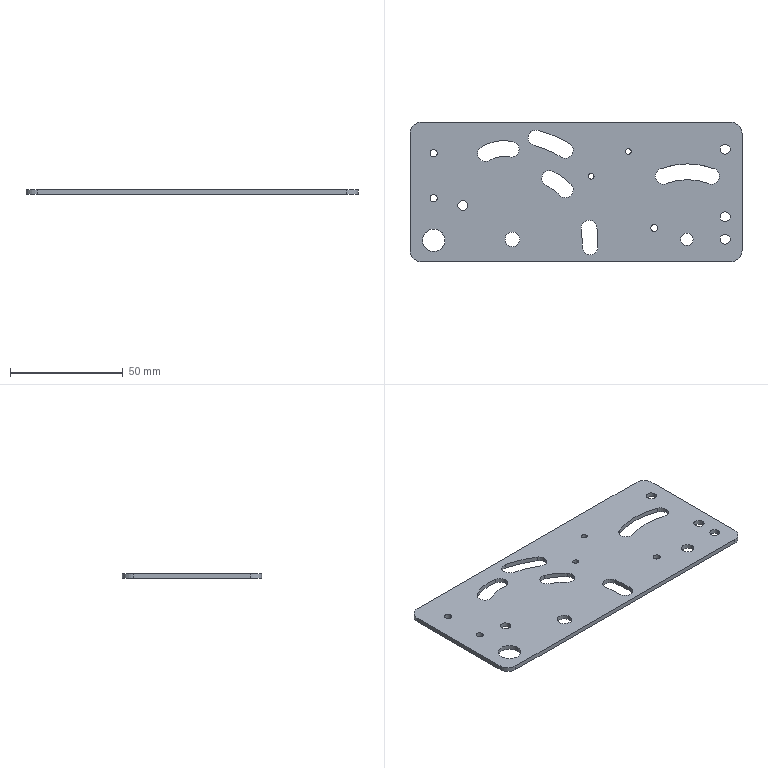Component | SolidWorks | CLS-MechanismBasePlate-1 | 1 solid | 60 faces | volume 16482 mm3 | cylinder 54 | plane 6 | commonest cylinder face diameters 7 x14 4.5 x8 3.2 x6 10 x6 2.5 x4 105.737 x2 119.737 x2 6.5 x2 | material 2.0 Galvanized Sheet Q235A